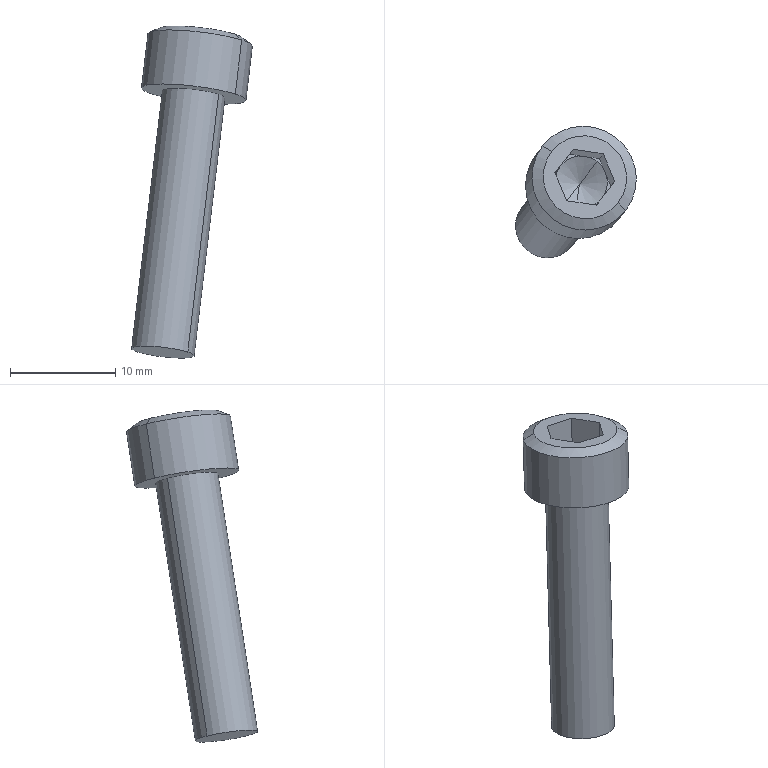Component | SolidWorks | MISUMI_MCSLC50-24-24_StandardCoupling-1_NEZI-1_MISUMI_MCSLC50-24-24_StandardCoupling-1 | 1 solid | 23 faces | box 11.49 x 12.48 x 31.59 mm | volume 1081 mm3 | plane 15 | cone 4 | cylinder 4 | commonest cylinder face diameters 10 x2 6 x2
STEP:
#1=COLOUR_RGB('',0.7922,0.8196,0.9333);
#2=FILL_AREA_STYLE_COLOUR('',#1);
#3=FILL_AREA_STYLE('',(#2));
#4=SURFACE_STYLE_FILL_AREA(#3);
#5=SURFACE_SIDE_STYLE('',(#4));
#6=SURFACE_STYLE_USAGE(.BOTH.,#5);
#7=PRESENTATION_STYLE_ASSIGNMENT((#6));
#8=CARTESIAN_POINT('',(-7.796,34.631,11.332));
#9=VERTEX_POINT('',#8);
#10=CARTESIAN_POINT('',(-7.848,34.563,11.406));
#11=VERTEX_POINT('',#10);
#12=CARTESIAN_POINT('',(-7.796,34.631,11.332));
#13=DIRECTION('',(-0.4626,-0.5959,0.6564));
#14=VECTOR('',#13,39.37);
#15=LINE('',#12,#14);
#16=EDGE_CURVE('',#9,#11,#15,.T.);
#17=ORIENTED_EDGE('',*,*,#16,.F.);
#18=CARTESIAN_POINT('',(-7.73,34.716,11.369));
#19=VERTEX_POINT('',#18);
#20=CARTESIAN_POINT('',(-7.796,34.631,11.332));
#21=DIRECTION('',(0.5799,0.747,0.3251));
#22=VECTOR('',#21,39.37);
#23=LINE('',#20,#22);
#24=EDGE_CURVE('',#9,#19,#23,.T.);
#25=ORIENTED_EDGE('',*,*,#24,.T.);
#26=CARTESIAN_POINT('',(-7.777,34.736,11.371));
#27=VERTEX_POINT('',#26);
#28=CARTESIAN_POINT('',(-7.789,34.64,11.388));
#29=DIRECTION('',(-0.1173,-0.1511,-0.9815));
#30=DIRECTION('',(0.6019,0.7754,-0.1912));
#31=AXIS2_PLACEMENT_3D('',#28,#29,#30);
#32=CIRCLE('',#31,0.09843);
#33=EDGE_CURVE('',#27,#19,#32,.T.);
#34=ORIENTED_EDGE('',*,*,#33,.F.);
#35=CARTESIAN_POINT('',(-7.867,34.7,11.388));
#36=VERTEX_POINT('',#35);
#37=CARTESIAN_POINT('',(-7.789,34.64,11.388));
#38=DIRECTION('',(-0.1173,-0.1511,-0.9815));
#39=DIRECTION('',(0.6019,0.7754,-0.1912));
#40=AXIS2_PLACEMENT_3D('',#37,#38,#39);
#41=CIRCLE('',#40,0.09843);
#42=EDGE_CURVE('',#36,#27,#41,.T.);
#43=ORIENTED_EDGE('',*,*,#42,.F.);
#44=CARTESIAN_POINT('',(-7.879,34.604,11.404));
#45=VERTEX_POINT('',#44);
#46=CARTESIAN_POINT('',(-7.789,34.64,11.388));
#47=DIRECTION('',(-0.1173,-0.1511,-0.9815));
#48=DIRECTION('',(0.6019,0.7754,-0.1912));
#49=AXIS2_PLACEMENT_3D('',#46,#47,#48);
#50=CIRCLE('',#49,0.09843);
#51=EDGE_CURVE('',#45,#36,#50,.T.);
#52=ORIENTED_EDGE('',*,*,#51,.F.);
#53=CARTESIAN_POINT('',(-7.789,34.64,11.388));
#54=DIRECTION('',(-0.1173,-0.1511,-0.9815));
#55=DIRECTION('',(0.6019,0.7754,-0.1912));
#56=AXIS2_PLACEMENT_3D('',#53,#54,#55);
#57=CIRCLE('',#56,0.09843);
#58=EDGE_CURVE('',#11,#45,#57,.T.);
#59=ORIENTED_EDGE('',*,*,#58,.F.);
#60=EDGE_LOOP('',(#17,#25,#34,#43,#52,#59));
#61=FACE_OUTER_BOUND('',#60,.T.);
#62=CARTESIAN_POINT('',(-3.179,40.579,49.975));
#63=DIRECTION('',(0.1173,0.1511,0.9815));
#64=DIRECTION('',(-0.6019,-0.7754,0.1912));
#65=AXIS2_PLACEMENT_3D('',#62,#63,#64);
#66=CONICAL_SURFACE('',#65,68.191,1.047);
#67=ADVANCED_FACE('',(#61),#66,.F.);
#68=CARTESIAN_POINT('',(-7.651,34.561,11.503));
#69=VERTEX_POINT('',#68);
#70=CARTESIAN_POINT('',(-7.899,34.754,11.503));
#71=VERTEX_POINT('',#70);
#72=CARTESIAN_POINT('',(-7.775,34.657,11.503));
#73=DIRECTION('',(0.1173,0.1511,0.9815));
#74=DIRECTION('',(-0.7899,0.6132,0.));
#75=AXIS2_PLACEMENT_3D('',#72,#73,#74);
#76=CIRCLE('',#75,0.1572);
#77=EDGE_CURVE('',#69,#71,#76,.T.);
#78=ORIENTED_EDGE('',*,*,#77,.F.);
#79=CARTESIAN_POINT('',(-7.622,34.533,11.481));
#80=VERTEX_POINT('',#79);
#81=CARTESIAN_POINT('',(-7.651,34.561,11.503));
#82=DIRECTION('',(0.6255,-0.6066,-0.4908));
#83=VECTOR('',#82,39.37);
#84=LINE('',#81,#83);
#85=EDGE_CURVE('',#69,#80,#84,.T.);
#86=ORIENTED_EDGE('',*,*,#85,.T.);
#87=CARTESIAN_POINT('',(-7.933,34.775,11.481));
#88=VERTEX_POINT('',#87);
#89=CARTESIAN_POINT('',(-7.778,34.654,11.481));
#90=DIRECTION('',(-0.1173,-0.1511,-0.9815));
#91=DIRECTION('',(-0.7899,0.6132,0.));
#92=AXIS2_PLACEMENT_3D('',#89,#90,#91);
#93=CIRCLE('',#92,0.1969);
#94=EDGE_CURVE('',#88,#80,#93,.T.);
#95=ORIENTED_EDGE('',*,*,#94,.F.);
#96=CARTESIAN_POINT('',(-7.899,34.754,11.503));
#97=DIRECTION('',(-0.7427,0.4555,-0.4908));
#98=VECTOR('',#97,39.37);
#99=LINE('',#96,#98);
#100=EDGE_CURVE('',#71,#88,#99,.T.);
#101=ORIENTED_EDGE('',*,*,#100,.F.);
#102=EDGE_LOOP('',(#78,#86,#95,#101));
#103=FACE_OUTER_BOUND('',#102,.T.);
#104=CARTESIAN_POINT('',(-7.775,34.657,11.503));
#105=DIRECTION('',(-0.1173,-0.1511,-0.9815));
#106=DIRECTION('',(-0.7899,0.6132,0.));
#107=AXIS2_PLACEMENT_3D('',#104,#105,#106);
#108=CONICAL_SURFACE('',#107,0.1572,1.047);
#109=ADVANCED_FACE('',(#103),#108,.T.);
#110=CARTESIAN_POINT('',(-7.647,34.502,11.279));
#111=VERTEX_POINT('',#110);
#112=CARTESIAN_POINT('',(-7.958,34.744,11.279));
#113=VERTEX_POINT('',#112);
#114=CARTESIAN_POINT('',(-7.802,34.623,11.279));
#115=DIRECTION('',(0.1173,0.1511,0.9815));
#116=DIRECTION('',(0.7899,-0.6132,-0.));
#117=AXIS2_PLACEMENT_3D('',#114,#115,#116);
#118=CIRCLE('',#117,0.1969);
#119=EDGE_CURVE('',#111,#113,#118,.T.);
#120=ORIENTED_EDGE('',*,*,#119,.T.);
#121=CARTESIAN_POINT('',(-7.931,34.778,11.503));
#122=DIRECTION('',(0.1173,0.1511,0.9815));
#123=VECTOR('',#122,39.37);
#124=LINE('',#121,#123);
#125=EDGE_CURVE('',#113,#88,#124,.T.);
#126=ORIENTED_EDGE('',*,*,#125,.T.);
#127=ORIENTED_EDGE('',*,*,#94,.T.);
#128=CARTESIAN_POINT('',(-7.62,34.537,11.503));
#129=DIRECTION('',(0.1173,0.1511,0.9815));
#130=VECTOR('',#129,39.37);
#131=LINE('',#128,#130);
#132=EDGE_CURVE('',#111,#80,#131,.T.);
#133=ORIENTED_EDGE('',*,*,#132,.F.);
#134=EDGE_LOOP('',(#120,#126,#127,#133));
#135=FACE_OUTER_BOUND('',#134,.T.);
#136=CARTESIAN_POINT('',(-7.775,34.657,11.503));
#137=DIRECTION('',(0.1173,0.1511,0.9815));
#138=DIRECTION('',(0.7899,-0.6132,-0.));
#139=AXIS2_PLACEMENT_3D('',#136,#137,#138);
#140=CYLINDRICAL_SURFACE('',#139,0.1969);
#141=ADVANCED_FACE('',(#135),#140,.T.);
#142=CARTESIAN_POINT('',(-7.824,34.402,10.312));
#143=VERTEX_POINT('',#142);
#144=CARTESIAN_POINT('',(-8.011,34.547,10.312));
#145=VERTEX_POINT('',#144);
#146=CARTESIAN_POINT('',(-7.918,34.474,10.312));
#147=DIRECTION('',(0.1173,0.1511,0.9815));
#148=DIRECTION('',(0.7899,-0.6132,0.));
#149=AXIS2_PLACEMENT_3D('',#146,#147,#148);
#150=CIRCLE('',#149,0.1181);
#151=EDGE_CURVE('',#143,#145,#150,.T.);
#152=ORIENTED_EDGE('',*,*,#151,.T.);
#153=CARTESIAN_POINT('',(-7.895,34.695,11.279));
#154=VERTEX_POINT('',#153);
#155=CARTESIAN_POINT('',(-7.869,34.73,11.503));
#156=DIRECTION('',(0.1173,0.1511,0.9815));
#157=VECTOR('',#156,39.37);
#158=LINE('',#155,#157);
#159=EDGE_CURVE('',#145,#154,#158,.T.);
#160=ORIENTED_EDGE('',*,*,#159,.T.);
#161=CARTESIAN_POINT('',(-7.709,34.55,11.279));
#162=VERTEX_POINT('',#161);
#163=CARTESIAN_POINT('',(-7.802,34.623,11.279));
#164=DIRECTION('',(0.1173,0.1511,0.9815));
#165=DIRECTION('',(0.7899,-0.6132,0.));
#166=AXIS2_PLACEMENT_3D('',#163,#164,#165);
#167=CIRCLE('',#166,0.1181);
#168=EDGE_CURVE('',#162,#154,#167,.T.);
#169=ORIENTED_EDGE('',*,*,#168,.F.);
#170=CARTESIAN_POINT('',(-7.682,34.585,11.503));
#171=DIRECTION('',(0.1173,0.1511,0.9815));
#172=VECTOR('',#171,39.37);
#173=LINE('',#170,#172);
#174=EDGE_CURVE('',#143,#162,#173,.T.);
#175=ORIENTED_EDGE('',*,*,#174,.F.);
#176=EDGE_LOOP('',(#152,#160,#169,#175));
#177=FACE_OUTER_BOUND('',#176,.T.);
#178=CARTESIAN_POINT('',(-7.775,34.657,11.503));
#179=DIRECTION('',(0.1173,0.1511,0.9815));
#180=DIRECTION('',(0.7899,-0.6132,0.));
#181=AXIS2_PLACEMENT_3D('',#178,#179,#180);
#182=CYLINDRICAL_SURFACE('',#181,0.1181);
#183=ADVANCED_FACE('',(#177),#182,.T.);
#184=CARTESIAN_POINT('',(-7.677,34.623,11.377));
#185=VERTEX_POINT('',#184);
#186=CARTESIAN_POINT('',(-7.699,34.676,11.371));
#187=VERTEX_POINT('',#186);
#188=CARTESIAN_POINT('',(-7.677,34.623,11.377));
#189=DIRECTION('',(-0.3832,0.9187,-0.09562));
#190=VECTOR('',#189,39.37);
#191=LINE('',#188,#190);
#192=EDGE_CURVE('',#185,#187,#191,.T.);
#193=ORIENTED_EDGE('',*,*,#192,.T.);
#194=CARTESIAN_POINT('',(-7.711,34.579,11.388));
#195=VERTEX_POINT('',#194);
#196=CARTESIAN_POINT('',(-7.789,34.64,11.388));
#197=DIRECTION('',(-0.1173,-0.1511,-0.9815));
#198=DIRECTION('',(0.6019,0.7754,-0.1912));
#199=AXIS2_PLACEMENT_3D('',#196,#197,#198);
#200=CIRCLE('',#199,0.09843);
#201=EDGE_CURVE('',#187,#195,#200,.T.);
#202=ORIENTED_EDGE('',*,*,#201,.T.);
#203=CARTESIAN_POINT('',(-7.746,34.535,11.398));
#204=DIRECTION('',(0.6019,0.7754,-0.1912));
#205=VECTOR('',#204,39.37);
#206=LINE('',#203,#205);
#207=EDGE_CURVE('',#195,#185,#206,.T.);
#208=ORIENTED_EDGE('',*,*,#207,.T.);
#209=EDGE_LOOP('',(#193,#202,#208));
#210=FACE_OUTER_BOUND('',#209,.T.);
#211=CARTESIAN_POINT('',(-7.789,34.64,11.388));
#212=DIRECTION('',(0.1173,0.1511,0.9815));
#213=DIRECTION('',(0.7899,-0.6132,-0.));
#214=AXIS2_PLACEMENT_3D('',#211,#212,#213);
#215=PLANE('',#214);
#216=ADVANCED_FACE('',(#210),#215,.T.);
#217=CARTESIAN_POINT('',(-7.746,34.535,11.398));
#218=VERTEX_POINT('',#217);
#219=CARTESIAN_POINT('',(-7.746,34.535,11.398));
#220=DIRECTION('',(0.6019,0.7754,-0.1912));
#221=VECTOR('',#220,39.37);
#222=LINE('',#219,#221);
#223=EDGE_CURVE('',#218,#195,#222,.T.);
#224=ORIENTED_EDGE('',*,*,#223,.T.);
#225=CARTESIAN_POINT('',(-7.802,34.543,11.404));
#226=VERTEX_POINT('',#225);
#227=CARTESIAN_POINT('',(-7.789,34.64,11.388));
#228=DIRECTION('',(-0.1173,-0.1511,-0.9815));
#229=DIRECTION('',(0.6019,0.7754,-0.1912));
#230=AXIS2_PLACEMENT_3D('',#227,#228,#229);
#231=CIRCLE('',#230,0.09843);
#232=EDGE_CURVE('',#195,#226,#231,.T.);
#233=ORIENTED_EDGE('',*,*,#232,.T.);
#234=CARTESIAN_POINT('',(-7.858,34.551,11.409));
#235=DIRECTION('',(0.985,-0.1434,-0.09562));
#236=VECTOR('',#235,39.37);
#237=LINE('',#234,#236);
#238=EDGE_CURVE('',#226,#218,#237,.T.);
#239=ORIENTED_EDGE('',*,*,#238,.T.);
#240=EDGE_LOOP('',(#224,#233,#239));
#241=FACE_OUTER_BOUND('',#240,.T.);
#242=CARTESIAN_POINT('',(-7.789,34.64,11.388));
#243=DIRECTION('',(0.1173,0.1511,0.9815));
#244=DIRECTION('',(0.7899,-0.6132,-0.));
#245=AXIS2_PLACEMENT_3D('',#242,#243,#244);
#246=PLANE('',#245);
#247=ADVANCED_FACE('',(#241),#246,.T.);
#248=CARTESIAN_POINT('',(-7.858,34.551,11.409));
#249=VERTEX_POINT('',#248);
#250=CARTESIAN_POINT('',(-7.858,34.551,11.409));
#251=DIRECTION('',(0.985,-0.1434,-0.09562));
#252=VECTOR('',#251,39.37);
#253=LINE('',#250,#252);
#254=EDGE_CURVE('',#249,#226,#253,.T.);
#255=ORIENTED_EDGE('',*,*,#254,.T.);
#256=CARTESIAN_POINT('',(-7.789,34.64,11.388));
#257=DIRECTION('',(-0.1173,-0.1511,-0.9815));
#258=DIRECTION('',(0.6019,0.7754,-0.1912));
#259=AXIS2_PLACEMENT_3D('',#256,#257,#258);
#260=CIRCLE('',#259,0.09843);
#261=EDGE_CURVE('',#226,#11,#260,.T.);
#262=ORIENTED_EDGE('',*,*,#261,.T.);
#263=ORIENTED_EDGE('',*,*,#58,.T.);
#264=CARTESIAN_POINT('',(-7.901,34.656,11.398));
#265=DIRECTION('',(0.3832,-0.9187,0.09562));
#266=VECTOR('',#265,39.37);
#267=LINE('',#264,#266);
#268=EDGE_CURVE('',#45,#249,#267,.T.);
#269=ORIENTED_EDGE('',*,*,#268,.T.);
#270=EDGE_LOOP('',(#255,#262,#263,#269));
#271=FACE_OUTER_BOUND('',#270,.T.);
#272=CARTESIAN_POINT('',(-7.789,34.64,11.388));
#273=DIRECTION('',(0.1173,0.1511,0.9815));
#274=DIRECTION('',(0.7899,-0.6132,-0.));
#275=AXIS2_PLACEMENT_3D('',#272,#273,#274);
#276=PLANE('',#275);
#277=ADVANCED_FACE('',(#271),#276,.T.);
#278=CARTESIAN_POINT('',(-7.901,34.656,11.398));
#279=VERTEX_POINT('',#278);
#280=CARTESIAN_POINT('',(-7.901,34.656,11.398));
#281=DIRECTION('',(0.3832,-0.9187,0.09562));
#282=VECTOR('',#281,39.37);
#283=LINE('',#280,#282);
#284=EDGE_CURVE('',#279,#45,#283,.T.);
#285=ORIENTED_EDGE('',*,*,#284,.T.);
#286=ORIENTED_EDGE('',*,*,#51,.T.);
#287=CARTESIAN_POINT('',(-7.833,34.744,11.377));
#288=DIRECTION('',(-0.6019,-0.7754,0.1912));
#289=VECTOR('',#288,39.37);
#290=LINE('',#287,#289);
#291=EDGE_CURVE('',#36,#279,#290,.T.);
#292=ORIENTED_EDGE('',*,*,#291,.T.);
#293=EDGE_LOOP('',(#285,#286,#292));
#294=FACE_OUTER_BOUND('',#293,.T.);
#295=CARTESIAN_POINT('',(-7.789,34.64,11.388));
#296=DIRECTION('',(0.1173,0.1511,0.9815));
#297=DIRECTION('',(0.7899,-0.6132,-0.));
#298=AXIS2_PLACEMENT_3D('',#295,#296,#297);
#299=PLANE('',#298);
#300=ADVANCED_FACE('',(#294),#299,.T.);
#301=CARTESIAN_POINT('',(-7.833,34.744,11.377));
#302=VERTEX_POINT('',#301);
#303=CARTESIAN_POINT('',(-7.833,34.744,11.377));
#304=DIRECTION('',(-0.6019,-0.7754,0.1912));
#305=VECTOR('',#304,39.37);
#306=LINE('',#303,#305);
#307=EDGE_CURVE('',#302,#36,#306,.T.);
#308=ORIENTED_EDGE('',*,*,#307,.T.);
#309=ORIENTED_EDGE('',*,*,#42,.T.);
#310=CARTESIAN_POINT('',(-7.721,34.728,11.366));
#311=DIRECTION('',(-0.985,0.1434,0.09562));
#312=VECTOR('',#311,39.37);
#313=LINE('',#310,#312);
#314=EDGE_CURVE('',#27,#302,#313,.T.);
#315=ORIENTED_EDGE('',*,*,#314,.T.);
#316=EDGE_LOOP('',(#308,#309,#315));
#317=FACE_OUTER_BOUND('',#316,.T.);
#318=CARTESIAN_POINT('',(-7.789,34.64,11.388));
#319=DIRECTION('',(0.1173,0.1511,0.9815));
#320=DIRECTION('',(0.7899,-0.6132,-0.));
#321=AXIS2_PLACEMENT_3D('',#318,#319,#320);
#322=PLANE('',#321);
#323=ADVANCED_FACE('',(#317),#322,.T.);
#324=CARTESIAN_POINT('',(-7.721,34.728,11.366));
#325=VERTEX_POINT('',#324);
#326=CARTESIAN_POINT('',(-7.721,34.728,11.366));
#327=DIRECTION('',(-0.985,0.1434,0.09562));
#328=VECTOR('',#327,39.37);
#329=LINE('',#326,#328);
#330=EDGE_CURVE('',#325,#27,#329,.T.);
#331=ORIENTED_EDGE('',*,*,#330,.T.);
#332=ORIENTED_EDGE('',*,*,#33,.T.);
#333=CARTESIAN_POINT('',(-7.789,34.64,11.388));
#334=DIRECTION('',(-0.1173,-0.1511,-0.9815));
#335=DIRECTION('',(0.6019,0.7754,-0.1912));
#336=AXIS2_PLACEMENT_3D('',#333,#334,#335);
#337=CIRCLE('',#336,0.09843);
#338=EDGE_CURVE('',#19,#187,#337,.T.);
#339=ORIENTED_EDGE('',*,*,#338,.T.);
#340=CARTESIAN_POINT('',(-7.677,34.623,11.377));
#341=DIRECTION('',(-0.3832,0.9187,-0.09562));
#342=VECTOR('',#341,39.37);
#343=LINE('',#340,#342);
#344=EDGE_CURVE('',#187,#325,#343,.T.);
#345=ORIENTED_EDGE('',*,*,#344,.T.);
#346=EDGE_LOOP('',(#331,#332,#339,#345));
#347=FACE_OUTER_BOUND('',#346,.T.);
#348=CARTESIAN_POINT('',(-7.789,34.64,11.388));
#349=DIRECTION('',(0.1173,0.1511,0.9815));
#350=DIRECTION('',(0.7899,-0.6132,-0.));
#351=AXIS2_PLACEMENT_3D('',#348,#349,#350);
#352=PLANE('',#351);
#353=ADVANCED_FACE('',(#347),#352,.T.);
#354=ORIENTED_EDGE('',*,*,#151,.F.);
#355=CARTESIAN_POINT('',(-7.918,34.474,10.312));
#356=DIRECTION('',(0.1173,0.1511,0.9815));
#357=DIRECTION('',(0.7899,-0.6132,0.));
#358=AXIS2_PLACEMENT_3D('',#355,#356,#357);
#359=CIRCLE('',#358,0.1181);
#360=EDGE_CURVE('',#145,#143,#359,.T.);
#361=ORIENTED_EDGE('',*,*,#360,.F.);
#362=EDGE_LOOP('',(#354,#361));
#363=FACE_OUTER_BOUND('',#362,.T.);
#364=CARTESIAN_POINT('',(-7.846,34.566,10.29));
#365=DIRECTION('',(0.1173,0.1511,0.9815));
#366=DIRECTION('',(0.7899,-0.6132,-0.));
#367=AXIS2_PLACEMENT_3D('',#364,#365,#366);
#368=PLANE('',#367);
#369=ADVANCED_FACE('',(#363),#368,.F.);
#370=ORIENTED_EDGE('',*,*,#159,.F.);
#371=ORIENTED_EDGE('',*,*,#360,.T.);
#372=ORIENTED_EDGE('',*,*,#174,.T.);
#373=CARTESIAN_POINT('',(-7.802,34.623,11.279));
#374=DIRECTION('',(0.1173,0.1511,0.9815));
#375=DIRECTION('',(0.7899,-0.6132,0.));
#376=AXIS2_PLACEMENT_3D('',#373,#374,#375);
#377=CIRCLE('',#376,0.1181);
#378=EDGE_CURVE('',#154,#162,#377,.T.);
#379=ORIENTED_EDGE('',*,*,#378,.F.);
#380=EDGE_LOOP('',(#370,#371,#372,#379));
#381=FACE_OUTER_BOUND('',#380,.T.);
#382=CARTESIAN_POINT('',(-7.775,34.657,11.503));
#383=DIRECTION('',(0.1173,0.1511,0.9815));
#384=DIRECTION('',(0.7899,-0.6132,0.));
#385=AXIS2_PLACEMENT_3D('',#382,#383,#384);
#386=CYLINDRICAL_SURFACE('',#385,0.1181);
#387=ADVANCED_FACE('',(#381),#386,.T.);
#388=ORIENTED_EDGE('',*,*,#119,.F.);
#389=CARTESIAN_POINT('',(-7.802,34.623,11.279));
#390=DIRECTION('',(0.1173,0.1511,0.9815));
#391=DIRECTION('',(0.7899,-0.6132,-0.));
#392=AXIS2_PLACEMENT_3D('',#389,#390,#391);
#393=CIRCLE('',#392,0.1969);
#394=EDGE_CURVE('',#113,#111,#393,.T.);
#395=ORIENTED_EDGE('',*,*,#394,.F.);
#396=EDGE_LOOP('',(#388,#395));
#397=FACE_OUTER_BOUND('',#396,.T.);
#398=ORIENTED_EDGE('',*,*,#168,.T.);
#399=ORIENTED_EDGE('',*,*,#378,.T.);
#400=EDGE_LOOP('',(#398,#399));
#401=FACE_BOUND('',#400,.T.);
#402=CARTESIAN_POINT('',(-7.731,34.714,11.256));
#403=DIRECTION('',(0.1173,0.1511,0.9815));
#404=DIRECTION('',(0.7899,-0.6132,-0.));
#405=AXIS2_PLACEMENT_3D('',#402,#403,#404);
#406=PLANE('',#405);
#407=ADVANCED_FACE('',(#397,#401),#406,.F.);
#408=ORIENTED_EDGE('',*,*,#125,.F.);
#409=ORIENTED_EDGE('',*,*,#394,.T.);
#410=ORIENTED_EDGE('',*,*,#132,.T.);
#411=CARTESIAN_POINT('',(-7.778,34.654,11.481));
#412=DIRECTION('',(-0.1173,-0.1511,-0.9815));
#413=DIRECTION('',(-0.7899,0.6132,0.));
#414=AXIS2_PLACEMENT_3D('',#411,#412,#413);
#415=CIRCLE('',#414,0.1969);
#416=EDGE_CURVE('',#80,#88,#415,.T.);
#417=ORIENTED_EDGE('',*,*,#416,.T.);
#418=EDGE_LOOP('',(#408,#409,#410,#417));
#419=FACE_OUTER_BOUND('',#418,.T.);
#420=CARTESIAN_POINT('',(-7.775,34.657,11.503));
#421=DIRECTION('',(0.1173,0.1511,0.9815));
#422=DIRECTION('',(0.7899,-0.6132,-0.));
#423=AXIS2_PLACEMENT_3D('',#420,#421,#422);
#424=CYLINDRICAL_SURFACE('',#423,0.1969);
#425=ADVANCED_FACE('',(#419),#424,.T.);
#426=CARTESIAN_POINT('',(-7.775,34.657,11.503));
#427=DIRECTION('',(0.1173,0.1511,0.9815));
#428=DIRECTION('',(-0.7899,0.6132,0.));
#429=AXIS2_PLACEMENT_3D('',#426,#427,#428);
#430=CIRCLE('',#429,0.1572);
#431=EDGE_CURVE('',#71,#69,#430,.T.);
#432=ORIENTED_EDGE('',*,*,#431,.T.);
#433=ORIENTED_EDGE('',*,*,#77,.T.);
#434=EDGE_LOOP('',(#432,#433));
#435=FACE_OUTER_BOUND('',#434,.T.);
#436=CARTESIAN_POINT('',(-7.707,34.746,11.482));
#437=VERTEX_POINT('',#436);
#438=CARTESIAN_POINT('',(-7.819,34.762,11.493));
#439=VERTEX_POINT('',#438);
#440=CARTESIAN_POINT('',(-7.707,34.746,11.482));
#441=DIRECTION('',(-0.985,0.1434,0.09562));
#442=VECTOR('',#441,39.37);
#443=LINE('',#440,#442);
#444=EDGE_CURVE('',#437,#439,#443,.T.);
#445=ORIENTED_EDGE('',*,*,#444,.F.);
#446=CARTESIAN_POINT('',(-7.663,34.641,11.493));
#447=VERTEX_POINT('',#446);
#448=CARTESIAN_POINT('',(-7.663,34.641,11.493));
#449=DIRECTION('',(-0.3832,0.9187,-0.09562));
#450=VECTOR('',#449,39.37);
#451=LINE('',#448,#450);
#452=EDGE_CURVE('',#447,#437,#451,.T.);
#453=ORIENTED_EDGE('',*,*,#452,.F.);
#454=CARTESIAN_POINT('',(-7.732,34.553,11.514));
#455=VERTEX_POINT('',#454);
#456=CARTESIAN_POINT('',(-7.732,34.553,11.514));
#457=DIRECTION('',(0.6019,0.7754,-0.1912));
#458=VECTOR('',#457,39.37);
#459=LINE('',#456,#458);
#460=EDGE_CURVE('',#455,#447,#459,.T.);
#461=ORIENTED_EDGE('',*,*,#460,.F.);
#462=CARTESIAN_POINT('',(-7.844,34.569,11.525));
#463=VERTEX_POINT('',#462);
#464=CARTESIAN_POINT('',(-7.844,34.569,11.525));
#465=DIRECTION('',(0.985,-0.1434,-0.09562));
#466=VECTOR('',#465,39.37);
#467=LINE('',#464,#466);
#468=EDGE_CURVE('',#463,#455,#467,.T.);
#469=ORIENTED_EDGE('',*,*,#468,.F.);
#470=CARTESIAN_POINT('',(-7.887,34.674,11.514));
#471=VERTEX_POINT('',#470);
#472=CARTESIAN_POINT('',(-7.887,34.674,11.514));
#473=DIRECTION('',(0.3832,-0.9187,0.09562));
#474=VECTOR('',#473,39.37);
#475=LINE('',#472,#474);
#476=EDGE_CURVE('',#471,#463,#475,.T.);
#477=ORIENTED_EDGE('',*,*,#476,.F.);
#478=CARTESIAN_POINT('',(-7.819,34.762,11.493));
#479=DIRECTION('',(-0.6019,-0.7754,0.1912));
#480=VECTOR('',#479,39.37);
#481=LINE('',#478,#480);
#482=EDGE_CURVE('',#439,#471,#481,.T.);
#483=ORIENTED_EDGE('',*,*,#482,.F.);
#484=EDGE_LOOP('',(#445,#453,#461,#469,#477,#483));
#485=FACE_BOUND('',#484,.T.);
#486=CARTESIAN_POINT('',(-7.775,34.657,11.503));
#487=DIRECTION('',(-0.1173,-0.1511,-0.9815));
#488=DIRECTION('',(-0.7899,0.6132,0.));
#489=AXIS2_PLACEMENT_3D('',#486,#487,#488);
#490=PLANE('',#489);
#491=ADVANCED_FACE('',(#435,#485),#490,.F.);
#492=ORIENTED_EDGE('',*,*,#452,.T.);
#493=CARTESIAN_POINT('',(-7.721,34.728,11.366));
#494=DIRECTION('',(0.1173,0.1511,0.9815));
#495=VECTOR('',#494,39.37);
#496=LINE('',#493,#495);
#497=EDGE_CURVE('',#325,#437,#496,.T.);
#498=ORIENTED_EDGE('',*,*,#497,.F.);
#499=ORIENTED_EDGE('',*,*,#344,.F.);
#500=ORIENTED_EDGE('',*,*,#192,.F.);
#501=CARTESIAN_POINT('',(-7.677,34.623,11.377));
#502=DIRECTION('',(0.1173,0.1511,0.9815));
#503=VECTOR('',#502,39.37);
#504=LINE('',#501,#503);
#505=EDGE_CURVE('',#185,#447,#504,.T.);
#506=ORIENTED_EDGE('',*,*,#505,.T.);
#507=EDGE_LOOP('',(#492,#498,#499,#500,#506));
#508=FACE_OUTER_BOUND('',#507,.T.);
#509=CARTESIAN_POINT('',(-7.677,34.623,11.377));
#510=DIRECTION('',(0.9162,0.3649,-0.1656));
#511=DIRECTION('',(0.3832,-0.9187,0.09562));
#512=AXIS2_PLACEMENT_3D('',#509,#510,#511);
#513=PLANE('',#512);
#514=ADVANCED_FACE('',(#508),#513,.F.);
#515=ORIENTED_EDGE('',*,*,#460,.T.);
#516=ORIENTED_EDGE('',*,*,#505,.F.);
#517=ORIENTED_EDGE('',*,*,#207,.F.);
#518=ORIENTED_EDGE('',*,*,#223,.F.);
#519=CARTESIAN_POINT('',(-7.746,34.535,11.398));
#520=DIRECTION('',(0.1173,0.1511,0.9815));
#521=VECTOR('',#520,39.37);
#522=LINE('',#519,#521);
#523=EDGE_CURVE('',#218,#455,#522,.T.);
#524=ORIENTED_EDGE('',*,*,#523,.T.);
#525=EDGE_LOOP('',(#515,#516,#517,#518,#524));
#526=FACE_OUTER_BOUND('',#525,.T.);
#527=CARTESIAN_POINT('',(-7.746,34.535,11.398));
#528=DIRECTION('',(0.7899,-0.6132,-0.));
#529=DIRECTION('',(-0.1173,-0.1511,-0.9815));
#530=AXIS2_PLACEMENT_3D('',#527,#528,#529);
#531=PLANE('',#530);
#532=ADVANCED_FACE('',(#526),#531,.F.);
#533=ORIENTED_EDGE('',*,*,#468,.T.);
#534=ORIENTED_EDGE('',*,*,#523,.F.);
#535=ORIENTED_EDGE('',*,*,#238,.F.);
#536=ORIENTED_EDGE('',*,*,#254,.F.);
#537=CARTESIAN_POINT('',(-7.858,34.551,11.409));
#538=DIRECTION('',(0.1173,0.1511,0.9815));
#539=VECTOR('',#538,39.37);
#540=LINE('',#537,#539);
#541=EDGE_CURVE('',#249,#463,#540,.T.);
#542=ORIENTED_EDGE('',*,*,#541,.T.);
#543=EDGE_LOOP('',(#533,#534,#535,#536,#542));
#544=FACE_OUTER_BOUND('',#543,.T.);
#545=CARTESIAN_POINT('',(-7.858,34.551,11.409));
#546=DIRECTION('',(-0.1263,-0.9781,0.1656));
#547=DIRECTION('',(-0.985,0.1434,0.09562));
#548=AXIS2_PLACEMENT_3D('',#545,#546,#547);
#549=PLANE('',#548);
#550=ADVANCED_FACE('',(#544),#549,.F.);
#551=ORIENTED_EDGE('',*,*,#476,.T.);
#552=ORIENTED_EDGE('',*,*,#541,.F.);
#553=ORIENTED_EDGE('',*,*,#268,.F.);
#554=ORIENTED_EDGE('',*,*,#284,.F.);
#555=CARTESIAN_POINT('',(-7.901,34.656,11.398));
#556=DIRECTION('',(0.1173,0.1511,0.9815));
#557=VECTOR('',#556,39.37);
#558=LINE('',#555,#557);
#559=EDGE_CURVE('',#279,#471,#558,.T.);
#560=ORIENTED_EDGE('',*,*,#559,.T.);
#561=EDGE_LOOP('',(#551,#552,#553,#554,#560));
#562=FACE_OUTER_BOUND('',#561,.T.);
#563=CARTESIAN_POINT('',(-7.901,34.656,11.398));
#564=DIRECTION('',(-0.9162,-0.3649,0.1656));
#565=DIRECTION('',(-0.3832,0.9187,-0.09562));
#566=AXIS2_PLACEMENT_3D('',#563,#564,#565);
#567=PLANE('',#566);
#568=ADVANCED_FACE('',(#562),#567,.F.);
#569=ORIENTED_EDGE('',*,*,#482,.T.);
#570=ORIENTED_EDGE('',*,*,#559,.F.);
#571=ORIENTED_EDGE('',*,*,#291,.F.);
#572=ORIENTED_EDGE('',*,*,#307,.F.);
#573=CARTESIAN_POINT('',(-7.833,34.744,11.377));
#574=DIRECTION('',(0.1173,0.1511,0.9815));
#575=VECTOR('',#574,39.37);
#576=LINE('',#573,#575);
#577=EDGE_CURVE('',#302,#439,#576,.T.);
#578=ORIENTED_EDGE('',*,*,#577,.T.);
#579=EDGE_LOOP('',(#569,#570,#571,#572,#578));
#580=FACE_OUTER_BOUND('',#579,.T.);
#581=CARTESIAN_POINT('',(-7.833,34.744,11.377));
#582=DIRECTION('',(-0.7899,0.6132,0.));
#583=DIRECTION('',(0.1173,0.1511,0.9815));
#584=AXIS2_PLACEMENT_3D('',#581,#582,#583);
#585=PLANE('',#584);
#586=ADVANCED_FACE('',(#580),#585,.F.);
#587=ORIENTED_EDGE('',*,*,#444,.T.);
#588=ORIENTED_EDGE('',*,*,#577,.F.);
#589=ORIENTED_EDGE('',*,*,#314,.F.);
#590=ORIENTED_EDGE('',*,*,#330,.F.);
#591=ORIENTED_EDGE('',*,*,#497,.T.);
#592=EDGE_LOOP('',(#587,#588,#589,#590,#591));
#593=FACE_OUTER_BOUND('',#592,.T.);
#594=CARTESIAN_POINT('',(-7.721,34.728,11.366));
#595=DIRECTION('',(0.1263,0.9781,-0.1656));
#596=DIRECTION('',(0.985,-0.1434,-0.09562));
#597=AXIS2_PLACEMENT_3D('',#594,#595,#596);
#598=PLANE('',#597);
#599=ADVANCED_FACE('',(#593),#598,.F.);
#600=ORIENTED_EDGE('',*,*,#85,.F.);
#601=ORIENTED_EDGE('',*,*,#431,.F.);
#602=ORIENTED_EDGE('',*,*,#100,.T.);
#603=ORIENTED_EDGE('',*,*,#416,.F.);
#604=EDGE_LOOP('',(#600,#601,#602,#603));
#605=FACE_OUTER_BOUND('',#604,.T.);
#606=CARTESIAN_POINT('',(-7.775,34.657,11.503));
#607=DIRECTION('',(-0.1173,-0.1511,-0.9815));
#608=DIRECTION('',(-0.7899,0.6132,0.));
#609=AXIS2_PLACEMENT_3D('',#606,#607,#608);
#610=CONICAL_SURFACE('',#609,0.1572,1.047);
#611=ADVANCED_FACE('',(#605),#610,.T.);
#612=ORIENTED_EDGE('',*,*,#24,.F.);
#613=ORIENTED_EDGE('',*,*,#16,.T.);
#614=ORIENTED_EDGE('',*,*,#261,.F.);
#615=ORIENTED_EDGE('',*,*,#232,.F.);
#616=ORIENTED_EDGE('',*,*,#201,.F.);
#617=ORIENTED_EDGE('',*,*,#338,.F.);
#618=EDGE_LOOP('',(#612,#613,#614,#615,#616,#617));
#619=FACE_OUTER_BOUND('',#618,.T.);
#620=CARTESIAN_POINT('',(-3.179,40.579,49.975));
#621=DIRECTION('',(0.1173,0.1511,0.9815));
#622=DIRECTION('',(-0.6019,-0.7754,0.1912));
#623=AXIS2_PLACEMENT_3D('',#620,#621,#622);
#624=CONICAL_SURFACE('',#623,68.191,1.047);
#625=ADVANCED_FACE('',(#619),#624,.F.);
#626=CLOSED_SHELL('',(#67,#109,#141,#183,#216,#247,#277,#300,#323,#353,#369,#387,#407,#425,#491,#514,#532,#550,#568,#586,#599,#611,#625));
#627=MANIFOLD_SOLID_BREP('',#626);
#628=STYLED_ITEM('',(#7),#627);
#629=PRESENTATION_LAYER_ASSIGNMENT('','',(#628));
#630=CARTESIAN_POINT('',(0.,0.,0.));
#631=DIRECTION('',(0.,0.,1.));
#632=DIRECTION('',(1.,0.,0.));
#633=AXIS2_PLACEMENT_3D('',#630,#631,#632);
#634=(LENGTH_UNIT()NAMED_UNIT(*)SI_UNIT($,.METRE.));
#635=LENGTH_MEASURE_WITH_UNIT(LENGTH_MEASURE(0.0254),#634);
#636=DIMENSIONAL_EXPONENTS(1.,0.,0.,0.,0.,0.,0.);
#637=(CONVERSION_BASED_UNIT('',#635)LENGTH_UNIT()NAMED_UNIT(#636));
#638=UNCERTAINTY_MEASURE_WITH_UNIT(LENGTH_MEASURE(0.00001),#637,'','');
#639=(NAMED_UNIT(*)PLANE_ANGLE_UNIT()SI_UNIT($,.RADIAN.));
#640=(NAMED_UNIT(*)SI_UNIT($,.STERADIAN.)SOLID_ANGLE_UNIT());
#641=(GEOMETRIC_REPRESENTATION_CONTEXT(3)GLOBAL_UNCERTAINTY_ASSIGNED_CONTEXT((#638))GLOBAL_UNIT_ASSIGNED_CONTEXT((#637,#639,#640))REPRESENTATION_CONTEXT('',''));
#642=ADVANCED_BREP_SHAPE_REPRESENTATION('',(#627,#633),#641);
#643=(LENGTH_UNIT()NAMED_UNIT(*)SI_UNIT($,.METRE.));
#644=LENGTH_MEASURE_WITH_UNIT(LENGTH_MEASURE(0.0254),#643);
#645=DIMENSIONAL_EXPONENTS(1.,0.,0.,0.,0.,0.,0.);
#646=(CONVERSION_BASED_UNIT('',#644)LENGTH_UNIT()NAMED_UNIT(#645));
#647=UNCERTAINTY_MEASURE_WITH_UNIT(LENGTH_MEASURE(0.00001),#646,'','');
#648=(NAMED_UNIT(*)PLANE_ANGLE_UNIT()SI_UNIT($,.RADIAN.));
#649=(NAMED_UNIT(*)SI_UNIT($,.STERADIAN.)SOLID_ANGLE_UNIT());
#650=(GEOMETRIC_REPRESENTATION_CONTEXT(3)GLOBAL_UNCERTAINTY_ASSIGNED_CONTEXT((#647))GLOBAL_UNIT_ASSIGNED_CONTEXT((#646,#648,#649))REPRESENTATION_CONTEXT('',''));
#651=MECHANICAL_DESIGN_GEOMETRIC_PRESENTATION_REPRESENTATION('',(#628),#650);